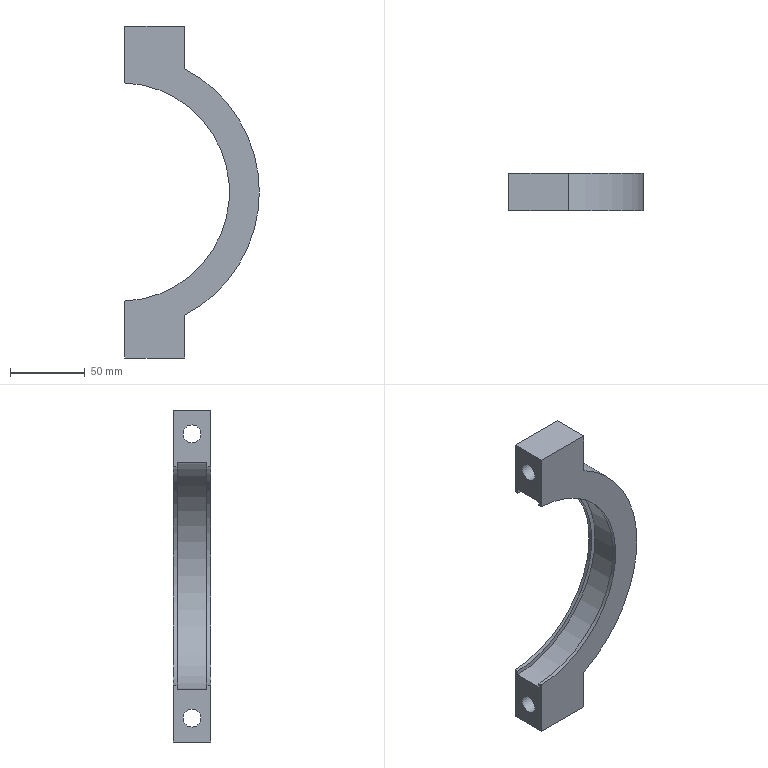Component | NX | STRAP_1 | 1 solid | 16 faces | volume 148015 mm3 | plane 10 | cylinder 6 | commonest cylinder face diameters 146 x2 12 x2 186 x1 152 x1